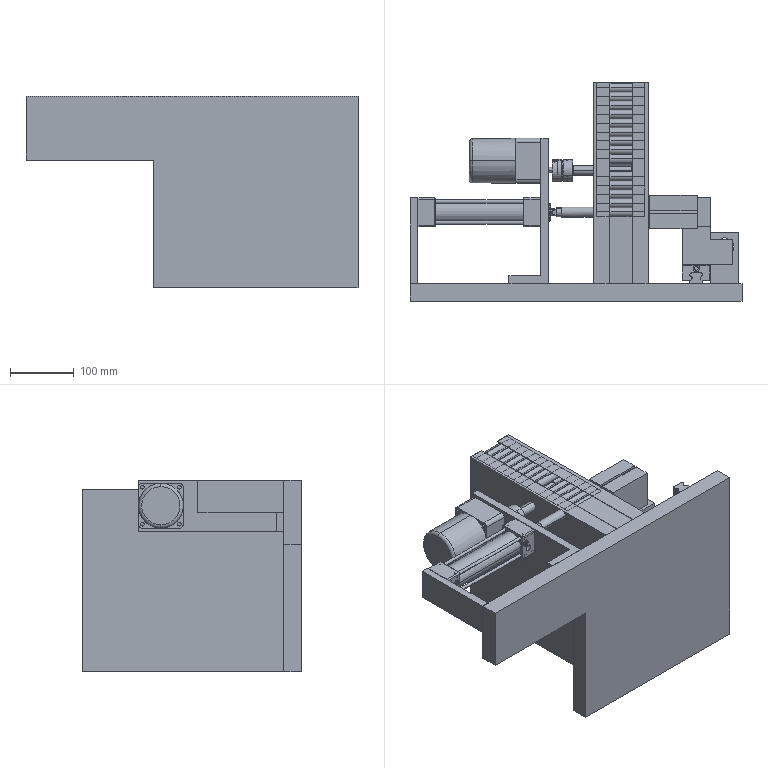Assembly | SolidWorks | mm | 65 component files | 65 solids | 2147 faces | box 520 x 342.5 x 300 mm | volume 10598929 mm3 | plane 986 | cylinder 783 | cone 294 | spline 82 | torus 2 | commonest cylinder face diameters 13.9 x72 11.9 x70 4 x62 6 x42 2 x39 1 x35 5 x32 10 x29
Bill of materials:
HZ022-3IK15RGN-C-3GN10K | 1 | SUS304 | Cylindrical body with a rounded rear end, joined to a square block housing. The block's front face has four corner through-holes and a small circular boss, and a stepped output shaft sticks out off-center from it. The overall shape looks like a gearmotor.
HZ022-A001-E001 | 1 | AL6061 | Thick rectangular block with a lengthwise slot or step along its top edge. Two small round holes sit near the top edge of the large face, and a small cylindrical pin sticks out sideways near the top. One side view shows a rectangular recess or pocket.
HZ022-A001-E002 | 1 | AL6061 | Thin flat plate of constant thickness with a stepped L-shaped outline: a rectangle with one corner notched out.
HZ022-A001-E003 | 1 | AL6061 | Angle bracket with an L-shaped cross-section. The longer leg has two round through-holes of slightly different sizes, offset toward one end.
HZ022-A001-E004 | 1 | S45C | Straight cylindrical shaft with six thin flat radial fins (vanes) evenly spaced around its middle section. One end has a short reduced-diameter step.
HZ022-A001-E005 | 1 | AL6061 | Plain rectangular bar or plate with no holes or cutouts.
HZ022-A001-E006 | 1 | S45C | Solid cylindrical pin with a chamfered (conical) taper at one end and a flat end face.
HZ022-A001-E007 | 1 | AL6061 | Rectangular flat plate or block with one large round through-hole set toward one end.
HZ022-A001-E009 | 1 | AL6061 | Stepped block with an L-shaped profile: a taller rectangular column on one side of a lower base section, plus a small notch or step in the top of the base.
HZ022-D14ToD10(D34x32L) | 1 | AL6061 | Cylindrical assembly-like body that looks like a disc-type shaft coupling. Two cylindrical hubs are separated by a thin central disc or spacer section with small axial pins. Each hub has a radial slit, and there is a counterbored hole for a transverse clamp. A central bore with a keyway runs through, and the end face has several axial holes.
HZ022-A001-E008 | 2 | AL6061 | Rectangular block with a stepped (rebated) profile on one side and a semicircular notch cut along one edge.
HZ022-HFP20 (1) | 1 | AL6061 | Complex fork-like part. Two upright parallel tabs, each with two round holes, rise from a central plate. The plate has slotted, oval and round holes and a shaped lower outline. Below it sits a cylindrical post ending in a stepped flange with grooves.
HZ022-HFP20 (2) | 1 | AL6061 | Rectangular block split by a central through-slot along most of its height, leaving two parallel jaws or plates. Small cylindrical pins cross the slot, and the faces carry several round holes and shallow longitudinal grooves.
HZ022-PenHolder1 | 35 |  | Straight thin-walled round tube with plain square-cut ends.
HZ022-HGH-20CAGuideRail | 1 | 45 | Long, slender straight bar with a constant profile. The cross-section has rounded side notches near the top and a flared, chamfered base. A single row of evenly spaced round holes runs through it along its length.
HZ022-HGH-20CASlider | 1 |  | Rectangular block with a shaped channel cut through its underside along its full length. The channel profile has rounded recesses on both sides. There are small notches on the top face, holes on the side and top faces, and a thin raised band or plate on one side.
HZ022-SC32x100S (1) | 1 | AL6061 | Cylindrical body between two square end blocks. Each block has four corner through holes and smaller side holes. A short hollow cylindrical boss sticks out from one end block, and the end face has a raised central circular feature with radial ribs or slots.
HZ022-SC32x100S (10) | 1 | AL6061 | Short thick-walled cylindrical sleeve or bushing with a through bore. One end is rounded or chamfered and the other end has a small chamfer.
HZ022-SC32x100S (11) | 1 | AL6061 | Short thick-walled cylindrical sleeve or bushing with a through bore. One end is rounded or chamfered and the other end has a small chamfer.
HZ022-SC32x100S (12) | 1 | AL6061 | Stepped cylindrical body. A larger-diameter end has a hexagonal socket recess, an external circumferential groove holding a rounded ring, and a thin flange. It tapers to a smaller-diameter cylindrical end.
HZ022-SC32x100S (13) | 1 | AL6061 | Stepped cylindrical body. A larger-diameter end has a hexagonal socket recess, an external circumferential groove holding a rounded ring, and a thin flange. It tapers to a smaller-diameter cylindrical end.
HZ022-SC32x100S (14) | 1 | AL6061 | Thin flat annular ring with six evenly spaced rectangular tabs around its outer edge. The tabs are bent out of the ring's plane.
HZ022-SC32x100S (15) | 1 | AL6061 | Thin flat annular ring with six evenly spaced rectangular tabs around its outer edge. The tabs are bent out of the ring's plane.
HZ022-SC32x100S (2) | 1 | AL6061 | Long slender stepped shaft. Near one end is a larger cylindrical section with several thin raised ribs or flanges. A long smaller-diameter shank leads to a reduced-diameter tip with a short flat or notch.
HZ022-SC32x100S (4) | 1 | AL6061 | Long, slender straight rod. One end has a short cylindrical tip slightly wider than the shaft. The other end has a larger cylindrical head with a short stepped neck and an open recess in its end face.
HZ022-SC32x100S (5) | 1 | AL6061 | Long, slender straight rod. One end has a short cylindrical tip slightly wider than the shaft. The other end has a larger cylindrical head with a short stepped neck and an open recess in its end face.
HZ022-SC32x100S (6) | 1 | AL6061 | Long, slender straight rod. One end has a short cylindrical tip slightly wider than the shaft. The other end has a larger cylindrical head with a short stepped neck and an open recess in its end face.
HZ022-SC32x100S (7) | 1 | AL6061 | Long, slender straight rod. One end has a short cylindrical tip slightly wider than the shaft. The other end has a larger cylindrical head with a short stepped neck and an open recess in its end face.
HZ022-SC32x100S (8) | 1 | AL6061 | Hollow cylindrical sleeve (tube) with a central through-bore. One end has a slight chamfer or taper. The other end has a small rounded edge.
HZ022-SC32x100S (9) | 1 | AL6061 | Hollow cylindrical sleeve (tube) with a central through-bore. One end has a slight chamfer or taper. The other end has a small rounded edge.
Mates:
1. coincident | HZ022-3IK15RGN-C-3GN10K-1 edge at (-57.556, 192.152, 910) dir (1, 0, 0) r 4.5 | HZ022-D14ToD10(D34x32L)-1 face at (-57.556, 208.366, 904.891) dir (1, 0, 0)
2. concentric | HZ022-A001-E001-1 face at (-7.556, 126.652, 927) dir (1, 0, 0) r 7 | HZ022-PenHolder1-1 face at (72.944, 126.652, 927) dir (-1, 0, 0) r 6.95
3. width | HZ022-PenHolder1-1 face at (-2.056, 126.652, 927) dir (-1, 0, 0) | HZ022-PenHolder1-1 face at (72.944, 126.652, 927) dir (1, 0, 0) | HZ022-A001-E001-1 face at (78.444, 79.652, 935) dir (1, 0, 0) | HZ022-A001-E001-1 face at (-7.556, 79.652, 935) dir (-1, 0, 0)
4. concentric | HZ022-SC32x100S-1/HZ022-SC32x100S (2)-1 face at (-53.94, 126.652, 927) dir (-1, 0, 0) r 5 | HZ022-A001-E006-1 face at (-2.556, 126.652, 927) dir (-1, 0, 0) r 7
5. coincident | HZ022-SC32x100S-1/HZ022-SC32x100S (2)-1 edge at (-64.556, 126.652, 927) dir (-1, 0, 0) r 5 | HZ022-A001-E006-1 face at (-64.556, 126.652, 927) dir (-1, 0, 0)
6. width | HZ022-HGH-20CASlider-1 face at (143.744, 28.118, 761) dir (1, 0, 0) | HZ022-HGH-20CASlider-1 face at (163.744, 29.176, 761) dir (-1, 0, 0) | HZ022-HGH-20CAGuideRail-1 face at (143.744, 29.176, 950) dir (-1, 0, 0) | HZ022-HGH-20CAGuideRail-1 face at (163.744, 28.118, 950) dir (1, 0, 0)
7. distance | HZ022-HGH-20CASlider-1 face at (141.744, 44.652, 761) dir (0, 1, 0) | HZ022-HGH-20CAGuideRail-1 face at (144.744, 14.652, 950) dir (0, -1, 0)
8. coincident | HZ022-HGH-20CASlider-1 face at (141.744, 44.652, 761) dir (0, 1, 0) | HZ022-A001-E009-1 face at (153.744, 44.652, 807.5) dir (0, -1, 0)
9. coincident | HZ022-HGH-20CASlider-1 face at (131.744, 43.652, 761) dir (-1, 0, 0) | HZ022-A001-E009-1 face at (131.744, 149.652, 747.5) dir (-1, 0, 0)
10. coincident | HZ022-HGH-20CASlider-1 face at (153.744, 32.152, 747.5) dir (0, 0, -1) | HZ022-A001-E009-1 face at (131.744, 149.652, 747.5) dir (0, 0, -1)
11. distance | HZ022-A001-E009-1 face at (131.744, 149.652, 747.5) dir (0, 0, -1) | HZ022-HFP20-1/HZ022-HFP20 (2)-1 face at (117.944, 126.652, 807.5) dir (0, 0, -1)
12. concentric | HZ022-A001-E001-1 face at (-12.056, 192.152, 910) dir (1, 0, 0) r 7.5 | HZ022-A001-E004-1 face at (78.444, 192.152, 910) dir (-1, 0, 0) r 7.5
13. coincident | HZ022-A001-E001-1 face at (78.444, 79.652, 935) dir (1, 0, 0) | HZ022-A001-E004-1 face at (78.444, 192.152, 910) dir (1, 0, 0)
14. coincident | HZ022-A001-E002-1 face at (-34.556, 14.652, 800) dir (0, 1, 0) | HZ022-A001-E003-1 face at (-89.556, 14.652, 870) dir (0, -1, 0)
15. concentric | HZ022-3IK15RGN-C-3GN10K-1 face at (-57.556, 192.152, 910) dir (-1, 0, 0) r 5 | HZ022-D14ToD10(D34x32L)-1 face at (-39.756, 192.152, 910) dir (1, 0, 0) r 7
16. distance | HZ022-A001-E003-1 face at (-77.556, 128.652, 910) dir (1, 0, 0) | HZ022-A001-E001-1 face at (-7.556, 79.652, 935) dir (-1, 0, 0)
17. coincident | HZ022-3IK15RGN-C-3GN10K-1 face at (-89.556, 236.152, 939) dir (1, 0, 0) | HZ022-A001-E003-1 face at (-89.556, 128.652, 910) dir (-1, 0, 0)
18. concentric | HZ022-3IK15RGN-C-3GN10K-1 face at (-86.556, 192.152, 910) dir (-1, 0, 0) r 15 | HZ022-A001-E003-1 face at (-77.555, 192.152, 910) dir (-1, 0, 0) r 15.5
19. concentric | HZ022-A001-E004-1 face at (78.444, 192.152, 910) dir (-1, 0, 0) r 7.5 | HZ022-D14ToD10(D34x32L)-1 face at (-39.756, 192.152, 910) dir (1, 0, 0) r 7
20. parallel | HZ022-3IK15RGN-C-3GN10K-1 face at (-128.556, 236.152, 945) dir (0, 0, 1) | HZ022-A001-E003-1 face at (-89.556, 14.652, 950) dir (0, 0, 1)
21. coincident | HZ022-A001-E003-1 face at (-89.556, 128.652, 910) dir (-1, 0, 0) | HZ022-SC32x100S-1/HZ022-SC32x100S (1)-1 face at (-89.556, 126.652, 927) dir (1, 0, 0)
22. concentric | HZ022-A001-E003-1 face at (-77.556, 126.652, 927) dir (-1, 0, 0) r 14 | HZ022-SC32x100S-1/HZ022-SC32x100S (1)-1 face at (-89.556, 126.652, 927) dir (1, 0, 0) r 14
23. parallel | HZ022-A001-E003-1 face at (-89.556, 14.652, 950) dir (0, 0, 1) | HZ022-SC32x100S-1/HZ022-SC32x100S (1)-1 face at (-89.556, 147.152, 949.5) dir (0, 0, 1)
24. coincident | HZ022-SC32x100S-1/HZ022-SC32x100S (1)-1 face at (-282.556, 126.652, 927) dir (-1, 0, 0) | HZ022-A001-E005-1 face at (-282.556, 81.902, 924.5) dir (1, 0, 0)
25. coincident | HZ022-SC32x100S-1/HZ022-SC32x100S (1)-1 face at (-282.556, 106.152, 949.5) dir (0, 0, 1) | HZ022-A001-E005-1 face at (-282.556, 149.152, 949.5) dir (0, 0, 1)
26. coincident | HZ022-SC32x100S-1/HZ022-SC32x100S (1)-1 face at (-282.556, 149.152, 947.5) dir (0, 1, 0) | HZ022-A001-E005-1 face at (-282.556, 149.152, 899.5) dir (0, 1, 0)
27. coincident | HZ022-A001-E002-1 face at (-34.556, 14.652, 800) dir (0, 1, 0) | HZ022-HGH-20CAGuideRail-1 face at (144.744, 14.652, 950) dir (0, -1, 0)
28. coincident | HZ022-A001-E002-1 face at (-294.556, 14.652, 950) dir (0, 0, 1) | HZ022-HGH-20CAGuideRail-1 face at (161.038, 31.382, 950) dir (0, 0, 1)
29. coincident | HZ022-HFP20-1/HZ022-HFP20 (2)-1 face at (131.744, 136.552, 876.3) dir (1, 0, 0) | HZ022-A001-E009-1 face at (131.744, 149.652, 747.5) dir (-1, 0, 0)
30. coincident | HZ022-A001-E002-1 face at (-294.556, 14.652, 950) dir (0, 0, 1) | HZ022-A001-E003-1 face at (-89.556, 14.652, 950) dir (0, 0, 1)
31. coincident | HZ022-A001-E002-1 face at (-34.556, 14.652, 800) dir (0, 1, 0) | HZ022-A001-E007-1 face at (220.744, 14.652, 784) dir (0, -1, 0)
32. distance | HZ022-HFP20-1/HZ022-A001-E008-2 face at (80.444, 152.902, 877) dir (-1, 0, 0) | HZ022-A001-E001-1 face at (78.444, 79.652, 935) dir (1, 0, 0)
33. coincident | HZ022-A001-E002-1 face at (-294.556, 14.652, 650) dir (-1, 0, 0) | HZ022-A001-E005-1 face at (-294.556, 81.902, 924.5) dir (-1, 0, 0)
34. distance | HZ022-A001-E007-1 face at (198.244, 54.652, 784) dir (0, 0, -1) | HZ022-A001-E002-1 face at (-294.556, 14.652, 950) dir (0, 0, 1)
35. coincident | HZ022-A001-E007-1 face at (175.744, 14.652, 784) dir (-1, 0, 0) | HZ022-A001-E009-1 face at (175.744, 149.652, 747.5) dir (1, 0, 0)
36. distance | HZ022-HFP20-1/HZ022-HFP20 (2)-1 face at (116.044, 149.152, 876.3) dir (0, 1, 0) | HZ022-A001-E009-1 face at (153.744, 149.652, 807.5) dir (0, 1, 0)
37. coincident | HZ022-A001-E002-1 face at (-34.556, 14.652, 800) dir (0, 1, 0) | HZ022-A001-E001-1 face at (-2.556, 14.652, 935) dir (0, -1, 0)
38. coincident | HZ022-HFP20 (1)-1 face at (-20.7, -16.05, 3.2) dir (-1, 0, 0) | HZ022-A001-E008-1 face at (-20.7, -2.25, 37.5) dir (1, 0, 0)
39. width | HZ022-A001-E008-1 face at (-0.7, -26.25, -37.5) dir (0, 0, -1) | HZ022-A001-E008-1 face at (-0.7, -26.25, 37.5) dir (0, 0, 1) | HZ022-HFP20 (1)-1 face at (0, 0, 6) dir (0, 0, 1) | HZ022-HFP20 (1)-1 face at (0, 0, -6) dir (0, 0, -1)
40. coincident | HZ022-HFP20 (1)-1 face at (-20.7, 16.05, -3.2) dir (-1, 0, 0) | HZ022-A001-E008-2 face at (-20.7, 2.25, -37.5) dir (1, 0, 0)
41. coincident | HZ022-A001-E008-1 face at (-0.7, -26.25, -37.5) dir (0, 0, -1) | HZ022-A001-E008-2 face at (-0.7, 26.25, -37.5) dir (0, 0, -1)
42. symmetric | HZ022-A001-E008-1 face at (-30.7, -2.25, 0) dir (0, 1, 0) | HZ022-A001-E008-2 face at (-30.7, 2.25, 0) dir (0, -1, 0) | HZ022-HFP20 plane at (0, 0, 0) dir (0, 1, 0)
43. distance | HZ022-A001-E008-2 face at (-30.7, 26.25, 0) dir (0, 1, 0) | HZ022-A001-E008-1 face at (-30.7, -26.25, 0) dir (0, -1, 0)
44. concentric | HZ022-A001-E008-2 face at (-50.7, 0, -37.5) dir (0, 0, 1) r 6.95 | HZ022-PenHolder1-1 face at (-50.7, 0, 37.5) dir (0, 0, -1) r 6.95
45. coincident | HZ022-A001-E008-2 face at (-0.7, 26.25, -37.5) dir (0, 0, -1) | HZ022-PenHolder1-1 face at (-50.7, 0, -37.5) dir (0, 0, -1)
46. concentric | HZ022-SC32x100S (1)-1 face at (-6.75, 0, 0) dir (1, 0, 0) r 6 | HZ022-SC32x100S (2)-1 face at (41.25, 0, 0) dir (1, 0, 0) r 6
47. distance | HZ022-SC32x100S (1)-1 face at (33.5, 12.1, 0) dir (1, 0, 0) | HZ022-SC32x100S (2)-1 face at (133.5, 7.242, -9.285) dir (-1, 0, 0)